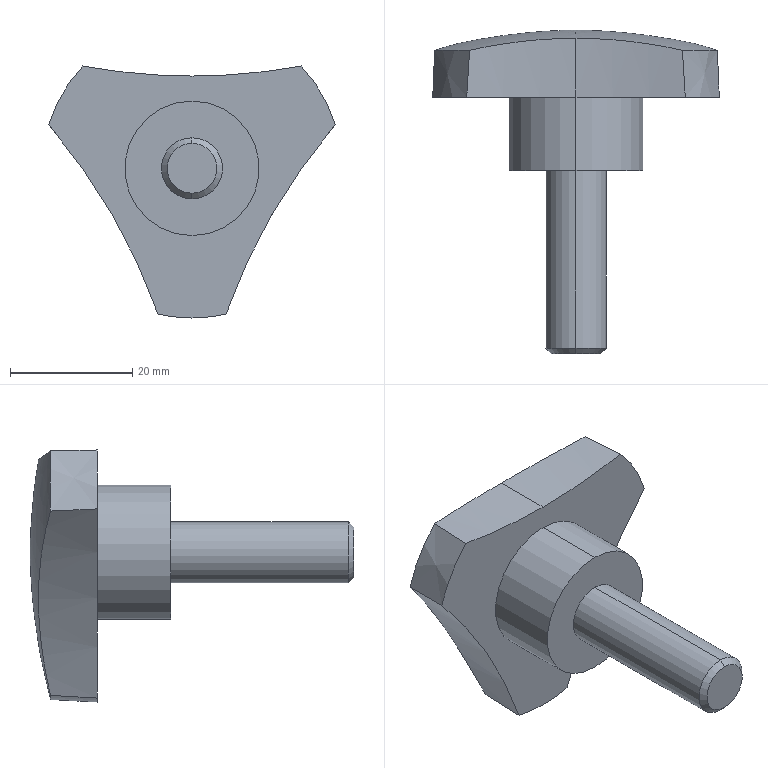Component | SolidWorks | NTM10-30-1 | 1 solid | 19 faces | box 47.54 x 53 x 48.6 mm | volume 18421 mm3 | cylinder 8 | cone 6 | plane 3 | spline 2 | commonest cylinder face diameters 196 x4 22 x2 10 x2 | material '-
STEP:
#1=COLOUR_RGB('',0.7922,0.8196,0.9333);
#2=FILL_AREA_STYLE_COLOUR('',#1);
#3=FILL_AREA_STYLE('',(#2));
#4=SURFACE_STYLE_FILL_AREA(#3);
#5=SURFACE_SIDE_STYLE('',(#4));
#6=SURFACE_STYLE_USAGE(.BOTH.,#5);
#7=PRESENTATION_STYLE_ASSIGNMENT((#6));
#8=CARTESIAN_POINT('',(0.,4.451,-0.));
#9=VERTEX_POINT('',#8);
#10=CARTESIAN_POINT('',(-0.,4.397,0.5946));
#11=VERTEX_POINT('',#10);
#12=CARTESIAN_POINT('',(0.,0.593,-0.05141));
#13=DIRECTION('',(1.,0.,0.));
#14=DIRECTION('',(0.,0.,1.));
#15=AXIS2_PLACEMENT_3D('',#12,#13,#14);
#16=CIRCLE('',#15,3.858);
#17=EDGE_CURVE('',#9,#11,#16,.T.);
#18=ORIENTED_EDGE('',*,*,#17,.F.);
#19=CARTESIAN_POINT('',(0.,4.319,-0.9488));
#20=VERTEX_POINT('',#19);
#21=CARTESIAN_POINT('',(0.,0.593,0.05141));
#22=DIRECTION('',(-1.,0.,-0.));
#23=DIRECTION('',(0.,0.,-1.));
#24=AXIS2_PLACEMENT_3D('',#21,#22,#23);
#25=CIRCLE('',#24,3.858);
#26=EDGE_CURVE('',#9,#20,#25,.T.);
#27=ORIENTED_EDGE('',*,*,#26,.T.);
#28=CARTESIAN_POINT('',(-0.2254,4.319,-0.9216));
#29=VERTEX_POINT('',#28);
#30=CARTESIAN_POINT('',(0.,4.319,-0.));
#31=DIRECTION('',(0.,-1.,0.));
#32=DIRECTION('',(1.,0.,-0.));
#33=AXIS2_PLACEMENT_3D('',#30,#31,#32);
#34=CIRCLE('',#33,0.9488);
#35=EDGE_CURVE('',#29,#20,#34,.T.);
#36=ORIENTED_EDGE('',*,*,#35,.F.);
#37=CARTESIAN_POINT('',(-0.9108,4.319,0.2656));
#38=VERTEX_POINT('',#37);
#39=CARTESIAN_POINT('',(-0.2254,4.319,-0.9216));
#40=CARTESIAN_POINT('',(-0.2638,4.345,-0.8146));
#41=CARTESIAN_POINT('',(-0.3071,4.364,-0.7091));
#42=CARTESIAN_POINT('',(-0.4033,4.39,-0.5012));
#43=CARTESIAN_POINT('',(-0.4563,4.397,-0.3989));
#44=CARTESIAN_POINT('',(-0.529,4.397,-0.273));
#45=CARTESIAN_POINT('',(-0.5439,4.396,-0.2478));
#46=CARTESIAN_POINT('',(-0.5741,4.395,-0.1981));
#47=CARTESIAN_POINT('',(-0.5894,4.393,-0.1735));
#48=CARTESIAN_POINT('',(-0.6362,4.389,-0.1003));
#49=CARTESIAN_POINT('',(-0.6683,4.384,-0.05246));
#50=CARTESIAN_POINT('',(-0.7675,4.364,0.08844));
#51=CARTESIAN_POINT('',(-0.8373,4.345,0.1788));
#52=CARTESIAN_POINT('',(-0.9108,4.319,0.2656));
#53=B_SPLINE_CURVE_WITH_KNOTS('',3,(#39,#40,#41,#42,#43,#44,#45,#46,#47,#48,#49,#50,#51,#52),.UNSPECIFIED.,.F.,.F.,(4,2,2,2,2,2,4),(0.,0.008783,0.01757,0.01976,0.02196,0.02635,0.03513),.UNSPECIFIED.);
#54=EDGE_CURVE('',#29,#38,#53,.T.);
#55=ORIENTED_EDGE('',*,*,#54,.T.);
#56=CARTESIAN_POINT('',(-0.6855,4.319,0.656));
#57=VERTEX_POINT('',#56);
#58=CARTESIAN_POINT('',(0.,4.319,-0.));
#59=DIRECTION('',(0.,-1.,0.));
#60=DIRECTION('',(1.,0.,-0.));
#61=AXIS2_PLACEMENT_3D('',#58,#59,#60);
#62=CIRCLE('',#61,0.9488);
#63=EDGE_CURVE('',#57,#38,#62,.T.);
#64=ORIENTED_EDGE('',*,*,#63,.F.);
#65=CARTESIAN_POINT('',(-0.6855,4.319,0.656));
#66=CARTESIAN_POINT('',(-0.5735,4.345,0.6358));
#67=CARTESIAN_POINT('',(-0.4605,4.364,0.6205));
#68=CARTESIAN_POINT('',(-0.232,4.39,0.5999));
#69=CARTESIAN_POINT('',(-0.1166,4.397,0.5946));
#70=CARTESIAN_POINT('',(-0.,4.397,0.5946));
#71=B_SPLINE_CURVE_WITH_KNOTS('',3,(#65,#66,#67,#68,#69,#70),.UNSPECIFIED.,.F.,.F.,(4,2,4),(-0.01759,-0.008795,0.),.UNSPECIFIED.);
#72=EDGE_CURVE('',#57,#11,#71,.T.);
#73=ORIENTED_EDGE('',*,*,#72,.T.);
#74=EDGE_LOOP('',(#18,#27,#36,#55,#64,#73));
#75=FACE_OUTER_BOUND('',#74,.T.);
#76=CARTESIAN_POINT('',(0.,4.451,0.));
#77=CARTESIAN_POINT('',(0.,4.451,0.));
#78=CARTESIAN_POINT('',(0.,4.451,-0.));
#79=CARTESIAN_POINT('',(0.,4.451,-0.));
#80=CARTESIAN_POINT('',(0.,4.447,-0.3209));
#81=CARTESIAN_POINT('',(-0.6418,4.447,-0.3209));
#82=CARTESIAN_POINT('',(-0.6418,4.447,0.3209));
#83=CARTESIAN_POINT('',(0.,4.447,0.3209));
#84=CARTESIAN_POINT('',(0.,4.403,-0.6388));
#85=CARTESIAN_POINT('',(-1.278,4.403,-0.6388));
#86=CARTESIAN_POINT('',(-1.278,4.403,0.6388));
#87=CARTESIAN_POINT('',(-0.,4.403,0.6388));
#88=CARTESIAN_POINT('',(0.,4.319,-0.9488));
#89=CARTESIAN_POINT('',(-1.898,4.319,-0.9488));
#90=CARTESIAN_POINT('',(-1.898,4.319,0.9488));
#91=CARTESIAN_POINT('',(-0.,4.319,0.9488));
#92=(BOUNDED_SURFACE()B_SPLINE_SURFACE(3,3,((#76,#77,#78,#79),(#80,#81,#82,#83),(#84,#85,#86,#87),(#88,#89,#90,#91)),.UNSPECIFIED.,.F.,.F.,.F.)B_SPLINE_SURFACE_WITH_KNOTS((4,4),(4,4),(0.,1.),(0.,1.),.UNSPECIFIED.)GEOMETRIC_REPRESENTATION_ITEM()RATIONAL_B_SPLINE_SURFACE(((1.,0.3333,0.3333,1.),(0.9948,0.3316,0.3316,0.9948),(0.9948,0.3316,0.3316,0.9948),(1.,0.3333,0.3333,1.)))REPRESENTATION_ITEM('')SURFACE());
#93=ADVANCED_FACE('',(#75),#92,.T.);
#94=CARTESIAN_POINT('',(0.,4.018,0.4331));
#95=VERTEX_POINT('',#94);
#96=CARTESIAN_POINT('',(0.,4.018,-0.4331));
#97=VERTEX_POINT('',#96);
#98=CARTESIAN_POINT('',(0.,4.018,-0.));
#99=DIRECTION('',(0.,1.,0.));
#100=DIRECTION('',(0.,0.,-1.));
#101=AXIS2_PLACEMENT_3D('',#98,#99,#100);
#102=CIRCLE('',#101,0.4331);
#103=EDGE_CURVE('',#95,#97,#102,.T.);
#104=ORIENTED_EDGE('',*,*,#103,.F.);
#105=CARTESIAN_POINT('',(0.,3.545,0.4331));
#106=VERTEX_POINT('',#105);
#107=CARTESIAN_POINT('',(0.,3.782,0.4331));
#108=DIRECTION('',(0.,-1.,0.));
#109=VECTOR('',#108,39.37);
#110=LINE('',#107,#109);
#111=EDGE_CURVE('',#95,#106,#110,.T.);
#112=ORIENTED_EDGE('',*,*,#111,.T.);
#113=CARTESIAN_POINT('',(0.,3.545,-0.4331));
#114=VERTEX_POINT('',#113);
#115=CARTESIAN_POINT('',(0.,3.545,-0.));
#116=DIRECTION('',(0.,1.,0.));
#117=DIRECTION('',(0.,0.,-1.));
#118=AXIS2_PLACEMENT_3D('',#115,#116,#117);
#119=CIRCLE('',#118,0.4331);
#120=EDGE_CURVE('',#106,#114,#119,.T.);
#121=ORIENTED_EDGE('',*,*,#120,.T.);
#122=CARTESIAN_POINT('',(0.,3.782,-0.4331));
#123=DIRECTION('',(0.,-1.,0.));
#124=VECTOR('',#123,39.37);
#125=LINE('',#122,#124);
#126=EDGE_CURVE('',#97,#114,#125,.T.);
#127=ORIENTED_EDGE('',*,*,#126,.F.);
#128=EDGE_LOOP('',(#104,#112,#121,#127));
#129=FACE_OUTER_BOUND('',#128,.T.);
#130=CARTESIAN_POINT('',(0.,3.782,-0.));
#131=DIRECTION('',(0.,-1.,0.));
#132=DIRECTION('',(0.,0.,-1.));
#133=AXIS2_PLACEMENT_3D('',#130,#131,#132);
#134=CYLINDRICAL_SURFACE('',#133,0.4331);
#135=ADVANCED_FACE('',(#129),#134,.T.);
#136=ORIENTED_EDGE('',*,*,#35,.T.);
#137=CARTESIAN_POINT('',(0.,4.018,-0.9646));
#138=VERTEX_POINT('',#137);
#139=CARTESIAN_POINT('',(0.,4.018,-0.9646));
#140=DIRECTION('',(-0.,-0.9986,-0.05234));
#141=VECTOR('',#140,39.37);
#142=LINE('',#139,#141);
#143=EDGE_CURVE('',#20,#138,#142,.T.);
#144=ORIENTED_EDGE('',*,*,#143,.T.);
#145=CARTESIAN_POINT('',(-0.219,4.018,-0.9394));
#146=VERTEX_POINT('',#145);
#147=CARTESIAN_POINT('',(0.,4.018,-0.));
#148=DIRECTION('',(-0.,-1.,-0.));
#149=DIRECTION('',(0.,0.,-1.));
#150=AXIS2_PLACEMENT_3D('',#147,#148,#149);
#151=CIRCLE('',#150,0.9646);
#152=EDGE_CURVE('',#146,#138,#151,.T.);
#153=ORIENTED_EDGE('',*,*,#152,.F.);
#154=CARTESIAN_POINT('',(-0.219,4.018,-0.9394));
#155=CARTESIAN_POINT('',(-0.2211,4.118,-0.9335));
#156=CARTESIAN_POINT('',(-0.2232,4.219,-0.9276));
#157=CARTESIAN_POINT('',(-0.2254,4.319,-0.9216));
#158=B_SPLINE_CURVE_WITH_KNOTS('',3,(#154,#155,#156,#157),.UNSPECIFIED.,.F.,.F.,(4,4),(0.,0.007674),.UNSPECIFIED.);
#159=EDGE_CURVE('',#146,#29,#158,.T.);
#160=ORIENTED_EDGE('',*,*,#159,.T.);
#161=EDGE_LOOP('',(#136,#144,#153,#160));
#162=FACE_OUTER_BOUND('',#161,.T.);
#163=CARTESIAN_POINT('',(0.,4.018,-0.));
#164=DIRECTION('',(-0.,-1.,-0.));
#165=DIRECTION('',(0.,0.,-1.));
#166=AXIS2_PLACEMENT_3D('',#163,#164,#165);
#167=CONICAL_SURFACE('',#166,0.9646,0.05236);
#168=ADVANCED_FACE('',(#162),#167,.T.);
#169=CARTESIAN_POINT('',(0.6855,4.319,0.656));
#170=VERTEX_POINT('',#169);
#171=CARTESIAN_POINT('',(-0.,4.397,0.5946));
#172=CARTESIAN_POINT('',(0.1166,4.397,0.5946));
#173=CARTESIAN_POINT('',(0.232,4.39,0.5999));
#174=CARTESIAN_POINT('',(0.4605,4.364,0.6205));
#175=CARTESIAN_POINT('',(0.5735,4.345,0.6358));
#176=CARTESIAN_POINT('',(0.6855,4.319,0.656));
#177=B_SPLINE_CURVE_WITH_KNOTS('',3,(#171,#172,#173,#174,#175,#176),.UNSPECIFIED.,.F.,.F.,(4,2,4),(0.,0.008795,0.01759),.UNSPECIFIED.);
#178=EDGE_CURVE('',#11,#170,#177,.T.);
#179=ORIENTED_EDGE('',*,*,#178,.F.);
#180=CARTESIAN_POINT('',(-0.,4.018,0.5946));
#181=VERTEX_POINT('',#180);
#182=CARTESIAN_POINT('',(-0.,4.018,0.5946));
#183=DIRECTION('',(0.,-1.,0.));
#184=VECTOR('',#183,39.37);
#185=LINE('',#182,#184);
#186=EDGE_CURVE('',#11,#181,#185,.T.);
#187=ORIENTED_EDGE('',*,*,#186,.T.);
#188=CARTESIAN_POINT('',(0.704,4.018,0.6594));
#189=VERTEX_POINT('',#188);
#190=CARTESIAN_POINT('',(-0.,4.018,4.453));
#191=DIRECTION('',(0.,1.,0.));
#192=DIRECTION('',(0.,0.,-1.));
#193=AXIS2_PLACEMENT_3D('',#190,#191,#192);
#194=CIRCLE('',#193,3.858);
#195=EDGE_CURVE('',#189,#181,#194,.T.);
#196=ORIENTED_EDGE('',*,*,#195,.F.);
#197=CARTESIAN_POINT('',(0.6855,4.319,0.656));
#198=CARTESIAN_POINT('',(0.6917,4.219,0.6571));
#199=CARTESIAN_POINT('',(0.6978,4.118,0.6582));
#200=CARTESIAN_POINT('',(0.704,4.018,0.6594));
#201=B_SPLINE_CURVE_WITH_KNOTS('',3,(#197,#198,#199,#200),.UNSPECIFIED.,.F.,.F.,(4,4),(0.,0.007674),.UNSPECIFIED.);
#202=EDGE_CURVE('',#170,#189,#201,.T.);
#203=ORIENTED_EDGE('',*,*,#202,.F.);
#204=EDGE_LOOP('',(#179,#187,#196,#203));
#205=FACE_OUTER_BOUND('',#204,.T.);
#206=CARTESIAN_POINT('',(-0.,4.018,4.453));
#207=DIRECTION('',(0.,-1.,0.));
#208=DIRECTION('',(0.,0.,-1.));
#209=AXIS2_PLACEMENT_3D('',#206,#207,#208);
#210=CYLINDRICAL_SURFACE('',#209,3.858);
#211=ADVANCED_FACE('',(#205),#210,.F.);
#212=CARTESIAN_POINT('',(0.,3.545,0.1969));
#213=VERTEX_POINT('',#212);
#214=CARTESIAN_POINT('',(0.,3.545,-0.1969));
#215=VERTEX_POINT('',#214);
#216=CARTESIAN_POINT('',(0.,3.545,-0.));
#217=DIRECTION('',(0.,1.,0.));
#218=DIRECTION('',(0.,0.,-1.));
#219=AXIS2_PLACEMENT_3D('',#216,#217,#218);
#220=CIRCLE('',#219,0.1969);
#221=EDGE_CURVE('',#213,#215,#220,.T.);
#222=ORIENTED_EDGE('',*,*,#221,.F.);
#223=CARTESIAN_POINT('',(0.,2.401,0.1969));
#224=VERTEX_POINT('',#223);
#225=CARTESIAN_POINT('',(0.,2.973,0.1969));
#226=DIRECTION('',(0.,-1.,0.));
#227=VECTOR('',#226,39.37);
#228=LINE('',#225,#227);
#229=EDGE_CURVE('',#213,#224,#228,.T.);
#230=ORIENTED_EDGE('',*,*,#229,.T.);
#231=CARTESIAN_POINT('',(0.,2.401,-0.1969));
#232=VERTEX_POINT('',#231);
#233=CARTESIAN_POINT('',(0.,2.401,-0.));
#234=DIRECTION('',(0.,1.,0.));
#235=DIRECTION('',(0.,0.,-1.));
#236=AXIS2_PLACEMENT_3D('',#233,#234,#235);
#237=CIRCLE('',#236,0.1969);
#238=EDGE_CURVE('',#224,#232,#237,.T.);
#239=ORIENTED_EDGE('',*,*,#238,.T.);
#240=CARTESIAN_POINT('',(0.,2.973,-0.1969));
#241=DIRECTION('',(0.,-1.,0.));
#242=VECTOR('',#241,39.37);
#243=LINE('',#240,#242);
#244=EDGE_CURVE('',#215,#232,#243,.T.);
#245=ORIENTED_EDGE('',*,*,#244,.F.);
#246=EDGE_LOOP('',(#222,#230,#239,#245));
#247=FACE_OUTER_BOUND('',#246,.T.);
#248=CARTESIAN_POINT('',(0.,2.973,-0.));
#249=DIRECTION('',(0.,-1.,0.));
#250=DIRECTION('',(0.,0.,-1.));
#251=AXIS2_PLACEMENT_3D('',#248,#249,#250);
#252=CYLINDRICAL_SURFACE('',#251,0.1969);
#253=ADVANCED_FACE('',(#247),#252,.T.);
#254=CARTESIAN_POINT('',(0.,2.364,0.1606));
#255=VERTEX_POINT('',#254);
#256=CARTESIAN_POINT('',(0.,2.364,-0.1606));
#257=VERTEX_POINT('',#256);
#258=CARTESIAN_POINT('',(0.,2.364,-0.));
#259=DIRECTION('',(0.,1.,0.));
#260=DIRECTION('',(0.,0.,1.));
#261=AXIS2_PLACEMENT_3D('',#258,#259,#260);
#262=CIRCLE('',#261,0.1606);
#263=EDGE_CURVE('',#255,#257,#262,.T.);
#264=ORIENTED_EDGE('',*,*,#263,.T.);
#265=CARTESIAN_POINT('',(0.,2.401,-0.1969));
#266=DIRECTION('',(0.,0.7071,-0.7071));
#267=VECTOR('',#266,39.37);
#268=LINE('',#265,#267);
#269=EDGE_CURVE('',#257,#232,#268,.T.);
#270=ORIENTED_EDGE('',*,*,#269,.T.);
#271=ORIENTED_EDGE('',*,*,#238,.F.);
#272=CARTESIAN_POINT('',(0.,2.401,0.1969));
#273=DIRECTION('',(0.,0.7071,0.7071));
#274=VECTOR('',#273,39.37);
#275=LINE('',#272,#274);
#276=EDGE_CURVE('',#255,#224,#275,.T.);
#277=ORIENTED_EDGE('',*,*,#276,.F.);
#278=EDGE_LOOP('',(#264,#270,#271,#277));
#279=FACE_OUTER_BOUND('',#278,.T.);
#280=CARTESIAN_POINT('',(0.,2.401,-0.));
#281=DIRECTION('',(0.,1.,0.));
#282=DIRECTION('',(0.,0.,1.));
#283=AXIS2_PLACEMENT_3D('',#280,#281,#282);
#284=CONICAL_SURFACE('',#283,0.1969,0.7854);
#285=ADVANCED_FACE('',(#279),#284,.T.);
#286=CARTESIAN_POINT('',(0.,4.018,-0.));
#287=DIRECTION('',(0.,1.,0.));
#288=DIRECTION('',(0.,0.,-1.));
#289=AXIS2_PLACEMENT_3D('',#286,#287,#288);
#290=CIRCLE('',#289,0.4331);
#291=EDGE_CURVE('',#97,#95,#290,.T.);
#292=ORIENTED_EDGE('',*,*,#291,.T.);
#293=ORIENTED_EDGE('',*,*,#103,.T.);
#294=EDGE_LOOP('',(#292,#293));
#295=FACE_BOUND('',#294,.T.);
#296=CARTESIAN_POINT('',(-0.923,4.018,0.28));
#297=VERTEX_POINT('',#296);
#298=CARTESIAN_POINT('',(-3.856,4.018,-2.226));
#299=DIRECTION('',(0.,1.,0.));
#300=DIRECTION('',(-0.,0.,-1.));
#301=AXIS2_PLACEMENT_3D('',#298,#299,#300);
#302=CIRCLE('',#301,3.858);
#303=EDGE_CURVE('',#297,#146,#302,.T.);
#304=ORIENTED_EDGE('',*,*,#303,.T.);
#305=ORIENTED_EDGE('',*,*,#152,.T.);
#306=CARTESIAN_POINT('',(0.219,4.018,-0.9394));
#307=VERTEX_POINT('',#306);
#308=CARTESIAN_POINT('',(0.,4.018,-0.));
#309=DIRECTION('',(-0.,-1.,-0.));
#310=DIRECTION('',(0.,0.,-1.));
#311=AXIS2_PLACEMENT_3D('',#308,#309,#310);
#312=CIRCLE('',#311,0.9646);
#313=EDGE_CURVE('',#138,#307,#312,.T.);
#314=ORIENTED_EDGE('',*,*,#313,.T.);
#315=CARTESIAN_POINT('',(0.923,4.018,0.28));
#316=VERTEX_POINT('',#315);
#317=CARTESIAN_POINT('',(3.856,4.018,-2.226));
#318=DIRECTION('',(0.,1.,0.));
#319=DIRECTION('',(0.,0.,-1.));
#320=AXIS2_PLACEMENT_3D('',#317,#318,#319);
#321=CIRCLE('',#320,3.858);
#322=EDGE_CURVE('',#307,#316,#321,.T.);
#323=ORIENTED_EDGE('',*,*,#322,.T.);
#324=CARTESIAN_POINT('',(0.,4.018,-0.));
#325=DIRECTION('',(0.,-1.,0.));
#326=DIRECTION('',(0.,0.,-1.));
#327=AXIS2_PLACEMENT_3D('',#324,#325,#326);
#328=CIRCLE('',#327,0.9646);
#329=EDGE_CURVE('',#316,#189,#328,.T.);
#330=ORIENTED_EDGE('',*,*,#329,.T.);
#331=ORIENTED_EDGE('',*,*,#195,.T.);
#332=CARTESIAN_POINT('',(-0.704,4.018,0.6594));
#333=VERTEX_POINT('',#332);
#334=CARTESIAN_POINT('',(-0.,4.018,4.453));
#335=DIRECTION('',(0.,1.,0.));
#336=DIRECTION('',(0.,0.,-1.));
#337=AXIS2_PLACEMENT_3D('',#334,#335,#336);
#338=CIRCLE('',#337,3.858);
#339=EDGE_CURVE('',#181,#333,#338,.T.);
#340=ORIENTED_EDGE('',*,*,#339,.T.);
#341=CARTESIAN_POINT('',(0.,4.018,-0.));
#342=DIRECTION('',(0.,-1.,0.));
#343=DIRECTION('',(0.,0.,-1.));
#344=AXIS2_PLACEMENT_3D('',#341,#342,#343);
#345=CIRCLE('',#344,0.9646);
#346=EDGE_CURVE('',#333,#297,#345,.T.);
#347=ORIENTED_EDGE('',*,*,#346,.T.);
#348=EDGE_LOOP('',(#304,#305,#314,#323,#330,#331,#340,#347));
#349=FACE_OUTER_BOUND('',#348,.T.);
#350=CARTESIAN_POINT('',(0.6988,4.018,-0.));
#351=DIRECTION('',(0.,-1.,0.));
#352=DIRECTION('',(0.,0.,-1.));
#353=AXIS2_PLACEMENT_3D('',#350,#351,#352);
#354=PLANE('',#353);
#355=ADVANCED_FACE('',(#295,#349),#354,.T.);
#356=ORIENTED_EDGE('',*,*,#111,.F.);
#357=ORIENTED_EDGE('',*,*,#291,.F.);
#358=ORIENTED_EDGE('',*,*,#126,.T.);
#359=CARTESIAN_POINT('',(0.,3.545,-0.));
#360=DIRECTION('',(0.,1.,0.));
#361=DIRECTION('',(0.,0.,-1.));
#362=AXIS2_PLACEMENT_3D('',#359,#360,#361);
#363=CIRCLE('',#362,0.4331);
#364=EDGE_CURVE('',#114,#106,#363,.T.);
#365=ORIENTED_EDGE('',*,*,#364,.T.);
#366=EDGE_LOOP('',(#356,#357,#358,#365));
#367=FACE_OUTER_BOUND('',#366,.T.);
#368=CARTESIAN_POINT('',(0.,3.782,-0.));
#369=DIRECTION('',(0.,-1.,0.));
#370=DIRECTION('',(0.,0.,-1.));
#371=AXIS2_PLACEMENT_3D('',#368,#369,#370);
#372=CYLINDRICAL_SURFACE('',#371,0.4331);
#373=ADVANCED_FACE('',(#367),#372,.T.);
#374=ORIENTED_EDGE('',*,*,#143,.F.);
#375=CARTESIAN_POINT('',(0.2254,4.319,-0.9216));
#376=VERTEX_POINT('',#375);
#377=CARTESIAN_POINT('',(0.,4.319,-0.));
#378=DIRECTION('',(0.,-1.,0.));
#379=DIRECTION('',(1.,0.,-0.));
#380=AXIS2_PLACEMENT_3D('',#377,#378,#379);
#381=CIRCLE('',#380,0.9488);
#382=EDGE_CURVE('',#20,#376,#381,.T.);
#383=ORIENTED_EDGE('',*,*,#382,.T.);
#384=CARTESIAN_POINT('',(0.2254,4.319,-0.9216));
#385=CARTESIAN_POINT('',(0.2232,4.219,-0.9276));
#386=CARTESIAN_POINT('',(0.2211,4.118,-0.9335));
#387=CARTESIAN_POINT('',(0.219,4.018,-0.9394));
#388=B_SPLINE_CURVE_WITH_KNOTS('',3,(#384,#385,#386,#387),.UNSPECIFIED.,.F.,.F.,(4,4),(0.,0.007674),.UNSPECIFIED.);
#389=EDGE_CURVE('',#376,#307,#388,.T.);
#390=ORIENTED_EDGE('',*,*,#389,.T.);
#391=ORIENTED_EDGE('',*,*,#313,.F.);
#392=EDGE_LOOP('',(#374,#383,#390,#391));
#393=FACE_OUTER_BOUND('',#392,.T.);
#394=CARTESIAN_POINT('',(0.,4.018,-0.));
#395=DIRECTION('',(-0.,-1.,-0.));
#396=DIRECTION('',(0.,0.,-1.));
#397=AXIS2_PLACEMENT_3D('',#394,#395,#396);
#398=CONICAL_SURFACE('',#397,0.9646,0.05236);
#399=ADVANCED_FACE('',(#393),#398,.T.);
#400=ORIENTED_EDGE('',*,*,#303,.F.);
#401=CARTESIAN_POINT('',(-0.9108,4.319,0.2656));
#402=CARTESIAN_POINT('',(-0.9149,4.219,0.2704));
#403=CARTESIAN_POINT('',(-0.919,4.118,0.2752));
#404=CARTESIAN_POINT('',(-0.923,4.018,0.28));
#405=B_SPLINE_CURVE_WITH_KNOTS('',3,(#401,#402,#403,#404),.UNSPECIFIED.,.F.,.F.,(4,4),(0.,0.007674),.UNSPECIFIED.);
#406=EDGE_CURVE('',#38,#297,#405,.T.);
#407=ORIENTED_EDGE('',*,*,#406,.F.);
#408=ORIENTED_EDGE('',*,*,#54,.F.);
#409=ORIENTED_EDGE('',*,*,#159,.F.);
#410=EDGE_LOOP('',(#400,#407,#408,#409));
#411=FACE_OUTER_BOUND('',#410,.T.);
#412=CARTESIAN_POINT('',(-3.856,4.018,-2.226));
#413=DIRECTION('',(0.,-1.,0.));
#414=DIRECTION('',(0.,0.,-1.));
#415=AXIS2_PLACEMENT_3D('',#412,#413,#414);
#416=CYLINDRICAL_SURFACE('',#415,3.858);
#417=ADVANCED_FACE('',(#411),#416,.F.);
#418=ORIENTED_EDGE('',*,*,#406,.T.);
#419=ORIENTED_EDGE('',*,*,#346,.F.);
#420=CARTESIAN_POINT('',(-0.704,4.018,0.6594));
#421=CARTESIAN_POINT('',(-0.6978,4.118,0.6582));
#422=CARTESIAN_POINT('',(-0.6917,4.219,0.6571));
#423=CARTESIAN_POINT('',(-0.6855,4.319,0.656));
#424=B_SPLINE_CURVE_WITH_KNOTS('',3,(#420,#421,#422,#423),.UNSPECIFIED.,.F.,.F.,(4,4),(0.,0.007674),.UNSPECIFIED.);
#425=EDGE_CURVE('',#333,#57,#424,.T.);
#426=ORIENTED_EDGE('',*,*,#425,.T.);
#427=ORIENTED_EDGE('',*,*,#63,.T.);
#428=EDGE_LOOP('',(#418,#419,#426,#427));
#429=FACE_OUTER_BOUND('',#428,.T.);
#430=CARTESIAN_POINT('',(0.,4.018,-0.));
#431=DIRECTION('',(0.,-1.,0.));
#432=DIRECTION('',(0.,0.,-1.));
#433=AXIS2_PLACEMENT_3D('',#430,#431,#432);
#434=CONICAL_SURFACE('',#433,0.9646,0.05236);
#435=ADVANCED_FACE('',(#429),#434,.T.);
#436=ORIENTED_EDGE('',*,*,#186,.F.);
#437=ORIENTED_EDGE('',*,*,#72,.F.);
#438=ORIENTED_EDGE('',*,*,#425,.F.);
#439=ORIENTED_EDGE('',*,*,#339,.F.);
#440=EDGE_LOOP('',(#436,#437,#438,#439));
#441=FACE_OUTER_BOUND('',#440,.T.);
#442=CARTESIAN_POINT('',(-0.,4.018,4.453));
#443=DIRECTION('',(0.,-1.,0.));
#444=DIRECTION('',(0.,0.,-1.));
#445=AXIS2_PLACEMENT_3D('',#442,#443,#444);
#446=CYLINDRICAL_SURFACE('',#445,3.858);
#447=ADVANCED_FACE('',(#441),#446,.F.);
#448=ORIENTED_EDGE('',*,*,#202,.T.);
#449=ORIENTED_EDGE('',*,*,#329,.F.);
#450=CARTESIAN_POINT('',(0.9108,4.319,0.2656));
#451=VERTEX_POINT('',#450);
#452=CARTESIAN_POINT('',(0.923,4.018,0.28));
#453=CARTESIAN_POINT('',(0.919,4.118,0.2752));
#454=CARTESIAN_POINT('',(0.9149,4.219,0.2704));
#455=CARTESIAN_POINT('',(0.9108,4.319,0.2656));
#456=B_SPLINE_CURVE_WITH_KNOTS('',3,(#452,#453,#454,#455),.UNSPECIFIED.,.F.,.F.,(4,4),(0.,0.007674),.UNSPECIFIED.);
#457=EDGE_CURVE('',#316,#451,#456,.T.);
#458=ORIENTED_EDGE('',*,*,#457,.T.);
#459=CARTESIAN_POINT('',(0.,4.319,-0.));
#460=DIRECTION('',(0.,-1.,0.));
#461=DIRECTION('',(1.,0.,-0.));
#462=AXIS2_PLACEMENT_3D('',#459,#460,#461);
#463=CIRCLE('',#462,0.9488);
#464=EDGE_CURVE('',#451,#170,#463,.T.);
#465=ORIENTED_EDGE('',*,*,#464,.T.);
#466=EDGE_LOOP('',(#448,#449,#458,#465));
#467=FACE_OUTER_BOUND('',#466,.T.);
#468=CARTESIAN_POINT('',(0.,4.018,-0.));
#469=DIRECTION('',(0.,-1.,0.));
#470=DIRECTION('',(0.,0.,-1.));
#471=AXIS2_PLACEMENT_3D('',#468,#469,#470);
#472=CONICAL_SURFACE('',#471,0.9646,0.05236);
#473=ADVANCED_FACE('',(#467),#472,.T.);
#474=ORIENTED_EDGE('',*,*,#322,.F.);
#475=ORIENTED_EDGE('',*,*,#389,.F.);
#476=CARTESIAN_POINT('',(0.9108,4.319,0.2656));
#477=CARTESIAN_POINT('',(0.8374,4.345,0.1788));
#478=CARTESIAN_POINT('',(0.7676,4.364,0.08859));
#479=CARTESIAN_POINT('',(0.6357,4.39,-0.0987));
#480=CARTESIAN_POINT('',(0.5736,4.397,-0.1958));
#481=CARTESIAN_POINT('',(0.5009,4.397,-0.3216));
#482=CARTESIAN_POINT('',(0.4866,4.396,-0.3471));
#483=CARTESIAN_POINT('',(0.4586,4.395,-0.3981));
#484=CARTESIAN_POINT('',(0.445,4.393,-0.4237));
#485=CARTESIAN_POINT('',(0.405,4.389,-0.5008));
#486=CARTESIAN_POINT('',(0.3796,4.384,-0.5525));
#487=CARTESIAN_POINT('',(0.3072,4.364,-0.7089));
#488=CARTESIAN_POINT('',(0.2638,4.345,-0.8145));
#489=CARTESIAN_POINT('',(0.2254,4.319,-0.9216));
#490=B_SPLINE_CURVE_WITH_KNOTS('',3,(#476,#477,#478,#479,#480,#481,#482,#483,#484,#485,#486,#487,#488,#489),.UNSPECIFIED.,.F.,.F.,(4,2,2,2,2,2,4),(0.,0.008783,0.01757,0.01976,0.02196,0.02635,0.03513),.UNSPECIFIED.);
#491=EDGE_CURVE('',#451,#376,#490,.T.);
#492=ORIENTED_EDGE('',*,*,#491,.F.);
#493=ORIENTED_EDGE('',*,*,#457,.F.);
#494=EDGE_LOOP('',(#474,#475,#492,#493));
#495=FACE_OUTER_BOUND('',#494,.T.);
#496=CARTESIAN_POINT('',(3.856,4.018,-2.226));
#497=DIRECTION('',(0.,-1.,0.));
#498=DIRECTION('',(0.,0.,-1.));
#499=AXIS2_PLACEMENT_3D('',#496,#497,#498);
#500=CYLINDRICAL_SURFACE('',#499,3.858);
#501=ADVANCED_FACE('',(#495),#500,.F.);
#502=ORIENTED_EDGE('',*,*,#364,.F.);
#503=ORIENTED_EDGE('',*,*,#120,.F.);
#504=EDGE_LOOP('',(#502,#503));
#505=FACE_OUTER_BOUND('',#504,.T.);
#506=CARTESIAN_POINT('',(0.,3.545,-0.));
#507=DIRECTION('',(0.,1.,0.));
#508=DIRECTION('',(0.,0.,-1.));
#509=AXIS2_PLACEMENT_3D('',#506,#507,#508);
#510=CIRCLE('',#509,0.1969);
#511=EDGE_CURVE('',#215,#213,#510,.T.);
#512=ORIENTED_EDGE('',*,*,#511,.T.);
#513=ORIENTED_EDGE('',*,*,#221,.T.);
#514=EDGE_LOOP('',(#512,#513));
#515=FACE_BOUND('',#514,.T.);
#516=CARTESIAN_POINT('',(0.2165,3.545,-0.));
#517=DIRECTION('',(0.,-1.,0.));
#518=DIRECTION('',(0.,0.,-1.));
#519=AXIS2_PLACEMENT_3D('',#516,#517,#518);
#520=PLANE('',#519);
#521=ADVANCED_FACE('',(#505,#515),#520,.T.);
#522=ORIENTED_EDGE('',*,*,#26,.F.);
#523=ORIENTED_EDGE('',*,*,#17,.T.);
#524=ORIENTED_EDGE('',*,*,#178,.T.);
#525=ORIENTED_EDGE('',*,*,#464,.F.);
#526=ORIENTED_EDGE('',*,*,#491,.T.);
#527=ORIENTED_EDGE('',*,*,#382,.F.);
#528=EDGE_LOOP('',(#522,#523,#524,#525,#526,#527));
#529=FACE_OUTER_BOUND('',#528,.T.);
#530=CARTESIAN_POINT('',(0.,4.451,-0.));
#531=CARTESIAN_POINT('',(-0.,4.451,-0.));
#532=CARTESIAN_POINT('',(-0.,4.451,0.));
#533=CARTESIAN_POINT('',(0.,4.451,0.));
#534=CARTESIAN_POINT('',(-0.,4.447,0.3209));
#535=CARTESIAN_POINT('',(0.6418,4.447,0.3209));
#536=CARTESIAN_POINT('',(0.6418,4.447,-0.3209));
#537=CARTESIAN_POINT('',(0.,4.447,-0.3209));
#538=CARTESIAN_POINT('',(-0.,4.403,0.6388));
#539=CARTESIAN_POINT('',(1.278,4.403,0.6388));
#540=CARTESIAN_POINT('',(1.278,4.403,-0.6388));
#541=CARTESIAN_POINT('',(0.,4.403,-0.6388));
#542=CARTESIAN_POINT('',(-0.,4.319,0.9488));
#543=CARTESIAN_POINT('',(1.898,4.319,0.9488));
#544=CARTESIAN_POINT('',(1.898,4.319,-0.9488));
#545=CARTESIAN_POINT('',(0.,4.319,-0.9488));
#546=(BOUNDED_SURFACE()B_SPLINE_SURFACE(3,3,((#530,#531,#532,#533),(#534,#535,#536,#537),(#538,#539,#540,#541),(#542,#543,#544,#545)),.UNSPECIFIED.,.F.,.F.,.T.)B_SPLINE_SURFACE_WITH_KNOTS((4,4),(4,4),(0.,1.),(0.,1.),.UNSPECIFIED.)GEOMETRIC_REPRESENTATION_ITEM()RATIONAL_B_SPLINE_SURFACE(((1.,0.3333,0.3333,1.),(0.9948,0.3316,0.3316,0.9948),(0.9948,0.3316,0.3316,0.9948),(1.,0.3333,0.3333,1.)))REPRESENTATION_ITEM('')SURFACE());
#547=ADVANCED_FACE('',(#529),#546,.T.);
#548=ORIENTED_EDGE('',*,*,#229,.F.);
#549=ORIENTED_EDGE('',*,*,#511,.F.);
#550=ORIENTED_EDGE('',*,*,#244,.T.);
#551=CARTESIAN_POINT('',(0.,2.401,-0.));
#552=DIRECTION('',(0.,1.,0.));
#553=DIRECTION('',(0.,0.,-1.));
#554=AXIS2_PLACEMENT_3D('',#551,#552,#553);
#555=CIRCLE('',#554,0.1969);
#556=EDGE_CURVE('',#232,#224,#555,.T.);
#557=ORIENTED_EDGE('',*,*,#556,.T.);
#558=EDGE_LOOP('',(#548,#549,#550,#557));
#559=FACE_OUTER_BOUND('',#558,.T.);
#560=CARTESIAN_POINT('',(0.,2.973,-0.));
#561=DIRECTION('',(0.,-1.,0.));
#562=DIRECTION('',(0.,0.,-1.));
#563=AXIS2_PLACEMENT_3D('',#560,#561,#562);
#564=CYLINDRICAL_SURFACE('',#563,0.1969);
#565=ADVANCED_FACE('',(#559),#564,.T.);
#566=ORIENTED_EDGE('',*,*,#269,.F.);
#567=CARTESIAN_POINT('',(0.,2.364,-0.));
#568=DIRECTION('',(0.,1.,0.));
#569=DIRECTION('',(0.,0.,1.));
#570=AXIS2_PLACEMENT_3D('',#567,#568,#569);
#571=CIRCLE('',#570,0.1606);
#572=EDGE_CURVE('',#257,#255,#571,.T.);
#573=ORIENTED_EDGE('',*,*,#572,.T.);
#574=ORIENTED_EDGE('',*,*,#276,.T.);
#575=ORIENTED_EDGE('',*,*,#556,.F.);
#576=EDGE_LOOP('',(#566,#573,#574,#575));
#577=FACE_OUTER_BOUND('',#576,.T.);
#578=CARTESIAN_POINT('',(0.,2.401,-0.));
#579=DIRECTION('',(0.,1.,0.));
#580=DIRECTION('',(0.,0.,1.));
#581=AXIS2_PLACEMENT_3D('',#578,#579,#580);
#582=CONICAL_SURFACE('',#581,0.1969,0.7854);
#583=ADVANCED_FACE('',(#577),#582,.T.);
#584=ORIENTED_EDGE('',*,*,#263,.F.);
#585=ORIENTED_EDGE('',*,*,#572,.F.);
#586=EDGE_LOOP('',(#584,#585));
#587=FACE_OUTER_BOUND('',#586,.T.);
#588=CARTESIAN_POINT('',(0.08031,2.364,-0.));
#589=DIRECTION('',(0.,-1.,0.));
#590=DIRECTION('',(0.,0.,-1.));
#591=AXIS2_PLACEMENT_3D('',#588,#589,#590);
#592=PLANE('',#591);
#593=ADVANCED_FACE('',(#587),#592,.T.);
#594=CLOSED_SHELL('',(#93,#135,#168,#211,#253,#285,#355,#373,#399,#417,#435,#447,#473,#501,#521,#547,#565,#583,#593));
#595=MANIFOLD_SOLID_BREP('',#594);
#596=STYLED_ITEM('',(#7),#595);
#597=PRESENTATION_LAYER_ASSIGNMENT('','',(#596));
#598=CARTESIAN_POINT('',(0.,0.,0.));
#599=DIRECTION('',(0.,0.,1.));
#600=DIRECTION('',(1.,0.,0.));
#601=AXIS2_PLACEMENT_3D('',#598,#599,#600);
#602=(LENGTH_UNIT()NAMED_UNIT(*)SI_UNIT($,.METRE.));
#603=LENGTH_MEASURE_WITH_UNIT(LENGTH_MEASURE(0.0254),#602);
#604=DIMENSIONAL_EXPONENTS(1.,0.,0.,0.,0.,0.,0.);
#605=(CONVERSION_BASED_UNIT('',#603)LENGTH_UNIT()NAMED_UNIT(#604));
#606=UNCERTAINTY_MEASURE_WITH_UNIT(LENGTH_MEASURE(0.00001),#605,'','');
#607=(NAMED_UNIT(*)PLANE_ANGLE_UNIT()SI_UNIT($,.RADIAN.));
#608=(NAMED_UNIT(*)SI_UNIT($,.STERADIAN.)SOLID_ANGLE_UNIT());
#609=(GEOMETRIC_REPRESENTATION_CONTEXT(3)GLOBAL_UNCERTAINTY_ASSIGNED_CONTEXT((#606))GLOBAL_UNIT_ASSIGNED_CONTEXT((#605,#607,#608))REPRESENTATION_CONTEXT('',''));
#610=ADVANCED_BREP_SHAPE_REPRESENTATION('',(#595,#601),#609);
#611=(LENGTH_UNIT()NAMED_UNIT(*)SI_UNIT($,.METRE.));
#612=LENGTH_MEASURE_WITH_UNIT(LENGTH_MEASURE(0.0254),#611);
#613=DIMENSIONAL_EXPONENTS(1.,0.,0.,0.,0.,0.,0.);
#614=(CONVERSION_BASED_UNIT('',#612)LENGTH_UNIT()NAMED_UNIT(#613));
#615=UNCERTAINTY_MEASURE_WITH_UNIT(LENGTH_MEASURE(0.00001),#614,'','');
#616=(NAMED_UNIT(*)PLANE_ANGLE_UNIT()SI_UNIT($,.RADIAN.));
#617=(NAMED_UNIT(*)SI_UNIT($,.STERADIAN.)SOLID_ANGLE_UNIT());
#618=(GEOMETRIC_REPRESENTATION_CONTEXT(3)GLOBAL_UNCERTAINTY_ASSIGNED_CONTEXT((#615))GLOBAL_UNIT_ASSIGNED_CONTEXT((#614,#616,#617))REPRESENTATION_CONTEXT('',''));
#619=MECHANICAL_DESIGN_GEOMETRIC_PRESENTATION_REPRESENTATION('',(#596),#618);